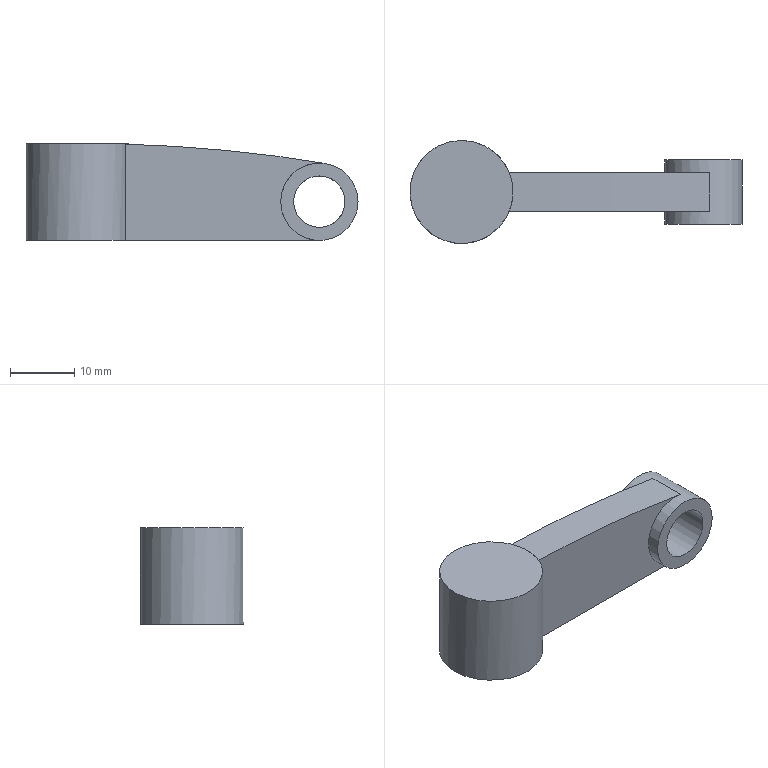Component | NX | CONNECTING_ROD_1 | 1 solid | 12 faces | box 51.54 x 16 x 15 mm | volume 4830 mm3 | plane 7 | cylinder 5 | commonest cylinder face diameters 16 x1 447 x1 12 x1 10 x1 8 x1
STEP:
#1=CARTESIAN_POINT('',(0.,0.,0.));
#2=DIRECTION('',(0.,0.,1.));
#3=DIRECTION('',(1.,0.,0.));
#4=AXIS2_PLACEMENT_3D('',#1,#2,#3);
#5=CARTESIAN_POINT('',(-285.764,8.,132.303));
#6=VERTEX_POINT('',#5);
#7=CARTESIAN_POINT('',(-285.764,0.,132.303));
#8=DIRECTION('',(0.,0.,-1.));
#9=DIRECTION('',(0.,1.,0.));
#10=AXIS2_PLACEMENT_3D('',#7,#8,#9);
#11=CIRCLE('',#10,8.);
#12=CARTESIAN_POINT('',(-285.764,0.,117.303));
#13=DIRECTION('',(0.,0.,1.));
#14=DIRECTION('',(0.,1.,0.));
#15=AXIS2_PLACEMENT_3D('',#12,#13,#14);
#16=CYLINDRICAL_SURFACE('',#15,8.);
#17=CARTESIAN_POINT('',(6.283,15.));
#18=DIRECTION('',(-1.,0.));
#19=VECTOR('',#18,1.);
#20=LINE('',#17,#19);
#21=(GEOMETRIC_REPRESENTATION_CONTEXT(2)PARAMETRIC_REPRESENTATION_CONTEXT()REPRESENTATION_CONTEXT('',''));
#22=DEFINITIONAL_REPRESENTATION('',(#20),#21);
#23=PCURVE('',#16,#22);
#24=CARTESIAN_POINT('',(-285.764,0.,132.303));
#25=DIRECTION('',(0.,0.,1.));
#26=DIRECTION('',(0.,1.,0.));
#27=AXIS2_PLACEMENT_3D('',#24,#25,#26);
#28=PLANE('',#27);
#29=CARTESIAN_POINT('',(8.,0.));
#30=CARTESIAN_POINT('',(8.,-13.856));
#31=CARTESIAN_POINT('',(-4.,-6.928));
#32=CARTESIAN_POINT('',(-16.,-0.));
#33=CARTESIAN_POINT('',(-4.,6.928));
#34=CARTESIAN_POINT('',(8.,13.856));
#35=CARTESIAN_POINT('',(8.,0.));
#36=(BOUNDED_CURVE()B_SPLINE_CURVE(2,(#29,#30,#31,#32,#33,#34,#35),.UNSPECIFIED.,.T.,.F.)B_SPLINE_CURVE_WITH_KNOTS((1,2,2,2,2,1),(-2.094,0.,2.094,4.189,6.283,8.378),.UNSPECIFIED.)CURVE()GEOMETRIC_REPRESENTATION_ITEM()RATIONAL_B_SPLINE_CURVE((1.,0.5,1.,0.5,1.,0.5,1.))REPRESENTATION_ITEM(''));
#37=(GEOMETRIC_REPRESENTATION_CONTEXT(2)PARAMETRIC_REPRESENTATION_CONTEXT()REPRESENTATION_CONTEXT('',''));
#38=DEFINITIONAL_REPRESENTATION('',(#36),#37);
#39=PCURVE('',#28,#38);
#40=SURFACE_CURVE('',#11,(#23,#39),.PCURVE_S1.);
#41=EDGE_CURVE('',#6,#6,#40,.T.);
#42=ORIENTED_EDGE('',*,*,#41,.T.);
#43=CARTESIAN_POINT('',(-285.764,8.,117.303));
#44=VERTEX_POINT('',#43);
#45=CARTESIAN_POINT('',(-285.764,8.,117.303));
#46=CARTESIAN_POINT('',(-285.764,8.,132.303));
#47=B_SPLINE_CURVE_WITH_KNOTS('',1,(#45,#46),.UNSPECIFIED.,.F.,.F.,(2,2),(0.,15.),.PIECEWISE_BEZIER_KNOTS.);
#48=CARTESIAN_POINT('',(0.,0.));
#49=DIRECTION('',(0.,1.));
#50=VECTOR('',#49,1.);
#51=LINE('',#48,#50);
#52=(GEOMETRIC_REPRESENTATION_CONTEXT(2)PARAMETRIC_REPRESENTATION_CONTEXT()REPRESENTATION_CONTEXT('',''));
#53=DEFINITIONAL_REPRESENTATION('',(#51),#52);
#54=PCURVE('',#16,#53);
#55=CARTESIAN_POINT('',(6.283,0.));
#56=DIRECTION('',(0.,1.));
#57=VECTOR('',#56,1.);
#58=LINE('',#55,#57);
#59=(GEOMETRIC_REPRESENTATION_CONTEXT(2)PARAMETRIC_REPRESENTATION_CONTEXT()REPRESENTATION_CONTEXT('',''));
#60=DEFINITIONAL_REPRESENTATION('',(#58),#59);
#61=PCURVE('',#16,#60);
#62=SEAM_CURVE('',#47,(#54,#61),.PCURVE_S1.);
#63=EDGE_CURVE('',#44,#6,#62,.T.);
#64=ORIENTED_EDGE('',*,*,#63,.F.);
#65=CARTESIAN_POINT('',(-278.348,-3.,117.303));
#66=VERTEX_POINT('',#65);
#67=CARTESIAN_POINT('',(-285.764,0.,117.303));
#68=DIRECTION('',(0.,0.,1.));
#69=DIRECTION('',(0.,1.,0.));
#70=AXIS2_PLACEMENT_3D('',#67,#68,#69);
#71=CIRCLE('',#70,8.);
#72=CARTESIAN_POINT('',(-0.,0.));
#73=DIRECTION('',(1.,0.));
#74=VECTOR('',#73,1.);
#75=LINE('',#72,#74);
#76=(GEOMETRIC_REPRESENTATION_CONTEXT(2)PARAMETRIC_REPRESENTATION_CONTEXT()REPRESENTATION_CONTEXT('',''));
#77=DEFINITIONAL_REPRESENTATION('',(#75),#76);
#78=PCURVE('',#16,#77);
#79=CARTESIAN_POINT('',(-285.764,0.,117.303));
#80=DIRECTION('',(0.,0.,-1.));
#81=DIRECTION('',(0.,-1.,0.));
#82=AXIS2_PLACEMENT_3D('',#79,#80,#81);
#83=PLANE('',#82);
#84=CARTESIAN_POINT('',(-8.,0.));
#85=CARTESIAN_POINT('',(-8.,13.856));
#86=CARTESIAN_POINT('',(4.,6.928));
#87=CARTESIAN_POINT('',(16.,0.));
#88=CARTESIAN_POINT('',(4.,-6.928));
#89=CARTESIAN_POINT('',(-8.,-13.856));
#90=CARTESIAN_POINT('',(-8.,0.));
#91=(BOUNDED_CURVE()B_SPLINE_CURVE(2,(#84,#85,#86,#87,#88,#89,#90),.UNSPECIFIED.,.T.,.F.)B_SPLINE_CURVE_WITH_KNOTS((1,2,2,2,2,1),(-2.094,0.,2.094,4.189,6.283,8.378),.UNSPECIFIED.)CURVE()GEOMETRIC_REPRESENTATION_ITEM()RATIONAL_B_SPLINE_CURVE((1.,0.5,1.,0.5,1.,0.5,1.))REPRESENTATION_ITEM(''));
#92=(GEOMETRIC_REPRESENTATION_CONTEXT(2)PARAMETRIC_REPRESENTATION_CONTEXT()REPRESENTATION_CONTEXT('',''));
#93=DEFINITIONAL_REPRESENTATION('',(#91),#92);
#94=PCURVE('',#83,#93);
#95=SURFACE_CURVE('',#71,(#78,#94),.PCURVE_S1.);
#96=EDGE_CURVE('',#44,#66,#95,.T.);
#97=ORIENTED_EDGE('',*,*,#96,.T.);
#98=CARTESIAN_POINT('',(-278.348,-3.,132.226));
#99=VERTEX_POINT('',#98);
#100=CARTESIAN_POINT('',(-278.348,-3.,117.303));
#101=DIRECTION('',(0.,0.,-1.));
#102=VECTOR('',#101,1.);
#103=LINE('',#100,#102);
#104=CARTESIAN_POINT('',(4.328,0.));
#105=DIRECTION('',(0.,-1.));
#106=VECTOR('',#105,1.);
#107=LINE('',#104,#106);
#108=(GEOMETRIC_REPRESENTATION_CONTEXT(2)PARAMETRIC_REPRESENTATION_CONTEXT()REPRESENTATION_CONTEXT('',''));
#109=DEFINITIONAL_REPRESENTATION('',(#107),#108);
#110=PCURVE('',#16,#109);
#111=CARTESIAN_POINT('',(-248.225,-3.,123.303));
#112=DIRECTION('',(0.,-1.,0.));
#113=DIRECTION('',(0.,0.,1.));
#114=AXIS2_PLACEMENT_3D('',#111,#112,#113);
#115=PLANE('',#114);
#116=CARTESIAN_POINT('',(-6.,30.123));
#117=DIRECTION('',(-1.,0.));
#118=VECTOR('',#117,1.);
#119=LINE('',#116,#118);
#120=(GEOMETRIC_REPRESENTATION_CONTEXT(2)PARAMETRIC_REPRESENTATION_CONTEXT()REPRESENTATION_CONTEXT('',''));
#121=DEFINITIONAL_REPRESENTATION('',(#119),#120);
#122=PCURVE('',#115,#121);
#123=SURFACE_CURVE('',#103,(#110,#122),.PCURVE_S1.);
#124=EDGE_CURVE('',#99,#66,#123,.T.);
#125=ORIENTED_EDGE('',*,*,#124,.F.);
#126=CARTESIAN_POINT('',(-278.348,3.,132.226));
#127=VERTEX_POINT('',#126);
#128=CARTESIAN_POINT('',(-278.348,-3.,132.226));
#129=CARTESIAN_POINT('',(-277.573,-1.083,132.205));
#130=CARTESIAN_POINT('',(-277.573,1.083,132.205));
#131=CARTESIAN_POINT('',(-278.348,3.,132.226));
#132=B_SPLINE_CURVE_WITH_KNOTS('',3,(#128,#129,#130,#131),.UNSPECIFIED.,.F.,.F.,(4,4),(0.,1.),.PIECEWISE_BEZIER_KNOTS.);
#133=CARTESIAN_POINT('',(4.328,14.923));
#134=CARTESIAN_POINT('',(5.097,14.923));
#135=B_SPLINE_CURVE_WITH_KNOTS('',1,(#133,#134),.UNSPECIFIED.,.F.,.F.,(2,2),(0.,1.),.PIECEWISE_BEZIER_KNOTS.);
#136=(GEOMETRIC_REPRESENTATION_CONTEXT(2)PARAMETRIC_REPRESENTATION_CONTEXT()REPRESENTATION_CONTEXT('',''));
#137=DEFINITIONAL_REPRESENTATION('',(#135),#136);
#138=PCURVE('',#16,#137);
#139=CARTESIAN_POINT('',(-284.225,3.,-91.197));
#140=DIRECTION('',(0.,-1.,0.));
#141=DIRECTION('',(0.,0.,1.));
#142=AXIS2_PLACEMENT_3D('',#139,#140,#141);
#143=CYLINDRICAL_SURFACE('',#142,223.5);
#144=CARTESIAN_POINT('',(6.257,6.));
#145=CARTESIAN_POINT('',(6.257,5.913));
#146=CARTESIAN_POINT('',(6.256,5.738));
#147=CARTESIAN_POINT('',(6.256,5.472));
#148=CARTESIAN_POINT('',(6.256,5.204));
#149=CARTESIAN_POINT('',(6.255,4.933));
#150=CARTESIAN_POINT('',(6.255,4.661));
#151=CARTESIAN_POINT('',(6.255,4.386));
#152=CARTESIAN_POINT('',(6.255,4.111));
#153=CARTESIAN_POINT('',(6.254,3.834));
#154=CARTESIAN_POINT('',(6.254,3.557));
#155=CARTESIAN_POINT('',(6.254,3.278));
#156=CARTESIAN_POINT('',(6.254,3.));
#157=CARTESIAN_POINT('',(6.254,2.722));
#158=CARTESIAN_POINT('',(6.254,2.443));
#159=CARTESIAN_POINT('',(6.254,2.166));
#160=CARTESIAN_POINT('',(6.255,1.889));
#161=CARTESIAN_POINT('',(6.255,1.614));
#162=CARTESIAN_POINT('',(6.255,1.339));
#163=CARTESIAN_POINT('',(6.255,1.067));
#164=CARTESIAN_POINT('',(6.256,0.7964));
#165=CARTESIAN_POINT('',(6.256,0.5281));
#166=CARTESIAN_POINT('',(6.256,0.2624));
#167=CARTESIAN_POINT('',(6.257,0.08712));
#168=CARTESIAN_POINT('',(6.257,0.));
#169=B_SPLINE_CURVE_WITH_KNOTS('',3,(#144,#145,#146,#147,#148,#149,#150,#151,#152,#153,#154,#155,#156,#157,#158,#159,#160,#161,#162,#163,#164,#165,#166,#167,#168),.UNSPECIFIED.,.F.,.F.,(4,1,1,1,1,1,1,1,1,1,1,1,1,1,1,1,1,1,1,1,1,1,4),(0.,0.04545,0.09091,0.1364,0.1818,0.2273,0.2727,0.3182,0.3636,0.4091,0.4545,0.5,0.5455,0.5909,0.6364,0.6818,0.7273,0.7727,0.8182,0.8636,0.9091,0.9545,1.),.QUASI_UNIFORM_KNOTS.);
#170=(GEOMETRIC_REPRESENTATION_CONTEXT(2)PARAMETRIC_REPRESENTATION_CONTEXT()REPRESENTATION_CONTEXT('',''));
#171=DEFINITIONAL_REPRESENTATION('',(#169),#170);
#172=PCURVE('',#143,#171);
#173=SURFACE_CURVE('',#132,(#138,#172),.PCURVE_S1.);
#174=EDGE_CURVE('',#99,#127,#173,.T.);
#175=ORIENTED_EDGE('',*,*,#174,.T.);
#176=CARTESIAN_POINT('',(-278.348,3.,117.303));
#177=VERTEX_POINT('',#176);
#178=CARTESIAN_POINT('',(-278.348,3.,117.303));
#179=DIRECTION('',(0.,0.,-1.));
#180=VECTOR('',#179,1.);
#181=LINE('',#178,#180);
#182=CARTESIAN_POINT('',(5.097,0.));
#183=DIRECTION('',(0.,-1.));
#184=VECTOR('',#183,1.);
#185=LINE('',#182,#184);
#186=(GEOMETRIC_REPRESENTATION_CONTEXT(2)PARAMETRIC_REPRESENTATION_CONTEXT()REPRESENTATION_CONTEXT('',''));
#187=DEFINITIONAL_REPRESENTATION('',(#185),#186);
#188=PCURVE('',#16,#187);
#189=CARTESIAN_POINT('',(-248.225,3.,123.303));
#190=DIRECTION('',(0.,-1.,0.));
#191=DIRECTION('',(0.,0.,1.));
#192=AXIS2_PLACEMENT_3D('',#189,#190,#191);
#193=PLANE('',#192);
#194=CARTESIAN_POINT('',(-6.,30.123));
#195=DIRECTION('',(-1.,0.));
#196=VECTOR('',#195,1.);
#197=LINE('',#194,#196);
#198=(GEOMETRIC_REPRESENTATION_CONTEXT(2)PARAMETRIC_REPRESENTATION_CONTEXT()REPRESENTATION_CONTEXT('',''));
#199=DEFINITIONAL_REPRESENTATION('',(#197),#198);
#200=PCURVE('',#193,#199);
#201=SURFACE_CURVE('',#181,(#188,#200),.PCURVE_S1.);
#202=EDGE_CURVE('',#127,#177,#201,.T.);
#203=ORIENTED_EDGE('',*,*,#202,.T.);
#204=CARTESIAN_POINT('',(-285.764,0.,117.303));
#205=DIRECTION('',(0.,0.,1.));
#206=DIRECTION('',(0.,1.,0.));
#207=AXIS2_PLACEMENT_3D('',#204,#205,#206);
#208=CIRCLE('',#207,8.);
#209=CARTESIAN_POINT('',(-0.,0.));
#210=DIRECTION('',(1.,0.));
#211=VECTOR('',#210,1.);
#212=LINE('',#209,#211);
#213=(GEOMETRIC_REPRESENTATION_CONTEXT(2)PARAMETRIC_REPRESENTATION_CONTEXT()REPRESENTATION_CONTEXT('',''));
#214=DEFINITIONAL_REPRESENTATION('',(#212),#213);
#215=PCURVE('',#16,#214);
#216=CARTESIAN_POINT('',(-8.,0.));
#217=CARTESIAN_POINT('',(-8.,13.856));
#218=CARTESIAN_POINT('',(4.,6.928));
#219=CARTESIAN_POINT('',(16.,0.));
#220=CARTESIAN_POINT('',(4.,-6.928));
#221=CARTESIAN_POINT('',(-8.,-13.856));
#222=CARTESIAN_POINT('',(-8.,0.));
#223=(BOUNDED_CURVE()B_SPLINE_CURVE(2,(#216,#217,#218,#219,#220,#221,#222),.UNSPECIFIED.,.T.,.F.)B_SPLINE_CURVE_WITH_KNOTS((1,2,2,2,2,1),(-2.094,0.,2.094,4.189,6.283,8.378),.UNSPECIFIED.)CURVE()GEOMETRIC_REPRESENTATION_ITEM()RATIONAL_B_SPLINE_CURVE((1.,0.5,1.,0.5,1.,0.5,1.))REPRESENTATION_ITEM(''));
#224=(GEOMETRIC_REPRESENTATION_CONTEXT(2)PARAMETRIC_REPRESENTATION_CONTEXT()REPRESENTATION_CONTEXT('',''));
#225=DEFINITIONAL_REPRESENTATION('',(#223),#224);
#226=PCURVE('',#83,#225);
#227=SURFACE_CURVE('',#208,(#215,#226),.PCURVE_S1.);
#228=EDGE_CURVE('',#177,#44,#227,.T.);
#229=ORIENTED_EDGE('',*,*,#228,.T.);
#230=ORIENTED_EDGE('',*,*,#63,.T.);
#231=EDGE_LOOP('',(#42,#64,#97,#125,#175,#203,#229,#230));
#232=FACE_BOUND('',#231,.T.);
#233=ADVANCED_FACE('',(#232),#16,.T.);
#234=ORIENTED_EDGE('',*,*,#41,.F.);
#235=EDGE_LOOP('',(#234));
#236=FACE_BOUND('',#235,.T.);
#237=ADVANCED_FACE('',(#236),#28,.T.);
#238=CARTESIAN_POINT('',(-290.764,0.,117.303));
#239=VERTEX_POINT('',#238);
#240=CARTESIAN_POINT('',(-285.764,0.,117.303));
#241=DIRECTION('',(0.,0.,-1.));
#242=DIRECTION('',(-1.,-0.,0.));
#243=AXIS2_PLACEMENT_3D('',#240,#241,#242);
#244=CIRCLE('',#243,5.);
#245=CARTESIAN_POINT('',(0.,0.));
#246=DIRECTION('',(0.,1.));
#247=AXIS2_PLACEMENT_2D('',#245,#246);
#248=CIRCLE('',#247,5.);
#249=(GEOMETRIC_REPRESENTATION_CONTEXT(2)PARAMETRIC_REPRESENTATION_CONTEXT()REPRESENTATION_CONTEXT('',''));
#250=DEFINITIONAL_REPRESENTATION('',(#248),#249);
#251=PCURVE('',#83,#250);
#252=CARTESIAN_POINT('',(-285.764,0.,129.303));
#253=DIRECTION('',(0.,0.,-1.));
#254=DIRECTION('',(0.,-1.,0.));
#255=AXIS2_PLACEMENT_3D('',#252,#253,#254);
#256=CYLINDRICAL_SURFACE('',#255,5.);
#257=CARTESIAN_POINT('',(1.571,12.));
#258=DIRECTION('',(1.,0.));
#259=VECTOR('',#258,1.);
#260=LINE('',#257,#259);
#261=(GEOMETRIC_REPRESENTATION_CONTEXT(2)PARAMETRIC_REPRESENTATION_CONTEXT()REPRESENTATION_CONTEXT('',''));
#262=DEFINITIONAL_REPRESENTATION('',(#260),#261);
#263=PCURVE('',#256,#262);
#264=SURFACE_CURVE('',#244,(#251,#263),.PCURVE_S1.);
#265=EDGE_CURVE('',#239,#239,#264,.T.);
#266=ORIENTED_EDGE('',*,*,#265,.F.);
#267=EDGE_LOOP('',(#266));
#268=FACE_BOUND('',#267,.T.);
#269=ORIENTED_EDGE('',*,*,#228,.F.);
#270=CARTESIAN_POINT('',(-248.225,3.,117.303));
#271=VERTEX_POINT('',#270);
#272=CARTESIAN_POINT('',(-248.225,3.,117.303));
#273=DIRECTION('',(-1.,0.,0.));
#274=VECTOR('',#273,1.);
#275=LINE('',#272,#274);
#276=CARTESIAN_POINT('',(-3.,-37.539));
#277=DIRECTION('',(0.,1.));
#278=VECTOR('',#277,1.);
#279=LINE('',#276,#278);
#280=(GEOMETRIC_REPRESENTATION_CONTEXT(2)PARAMETRIC_REPRESENTATION_CONTEXT()REPRESENTATION_CONTEXT('',''));
#281=DEFINITIONAL_REPRESENTATION('',(#279),#280);
#282=PCURVE('',#83,#281);
#283=CARTESIAN_POINT('',(-6.,0.));
#284=DIRECTION('',(0.,1.));
#285=VECTOR('',#284,1.);
#286=LINE('',#283,#285);
#287=(GEOMETRIC_REPRESENTATION_CONTEXT(2)PARAMETRIC_REPRESENTATION_CONTEXT()REPRESENTATION_CONTEXT('',''));
#288=DEFINITIONAL_REPRESENTATION('',(#286),#287);
#289=PCURVE('',#193,#288);
#290=SURFACE_CURVE('',#275,(#282,#289),.PCURVE_S1.);
#291=EDGE_CURVE('',#271,#177,#290,.T.);
#292=ORIENTED_EDGE('',*,*,#291,.F.);
#293=CARTESIAN_POINT('',(-248.225,-3.,117.303));
#294=VERTEX_POINT('',#293);
#295=CARTESIAN_POINT('',(-248.225,3.,117.303));
#296=DIRECTION('',(0.,-1.,0.));
#297=VECTOR('',#296,1.);
#298=LINE('',#295,#297);
#299=CARTESIAN_POINT('',(-3.,-37.539));
#300=DIRECTION('',(1.,0.));
#301=VECTOR('',#300,1.);
#302=LINE('',#299,#301);
#303=(GEOMETRIC_REPRESENTATION_CONTEXT(2)PARAMETRIC_REPRESENTATION_CONTEXT()REPRESENTATION_CONTEXT('',''));
#304=DEFINITIONAL_REPRESENTATION('',(#302),#303);
#305=PCURVE('',#83,#304);
#306=CARTESIAN_POINT('',(-248.225,5.,123.303));
#307=DIRECTION('',(0.,-1.,0.));
#308=DIRECTION('',(0.,0.,1.));
#309=AXIS2_PLACEMENT_3D('',#306,#307,#308);
#310=CYLINDRICAL_SURFACE('',#309,6.);
#311=CARTESIAN_POINT('',(3.142,2.));
#312=DIRECTION('',(0.,1.));
#313=VECTOR('',#312,1.);
#314=LINE('',#311,#313);
#315=(GEOMETRIC_REPRESENTATION_CONTEXT(2)PARAMETRIC_REPRESENTATION_CONTEXT()REPRESENTATION_CONTEXT('',''));
#316=DEFINITIONAL_REPRESENTATION('',(#314),#315);
#317=PCURVE('',#310,#316);
#318=SURFACE_CURVE('',#298,(#305,#317),.PCURVE_S1.);
#319=EDGE_CURVE('',#271,#294,#318,.T.);
#320=ORIENTED_EDGE('',*,*,#319,.T.);
#321=CARTESIAN_POINT('',(-248.225,-3.,117.303));
#322=DIRECTION('',(-1.,0.,0.));
#323=VECTOR('',#322,1.);
#324=LINE('',#321,#323);
#325=CARTESIAN_POINT('',(3.,-37.539));
#326=DIRECTION('',(0.,1.));
#327=VECTOR('',#326,1.);
#328=LINE('',#325,#327);
#329=(GEOMETRIC_REPRESENTATION_CONTEXT(2)PARAMETRIC_REPRESENTATION_CONTEXT()REPRESENTATION_CONTEXT('',''));
#330=DEFINITIONAL_REPRESENTATION('',(#328),#329);
#331=PCURVE('',#83,#330);
#332=CARTESIAN_POINT('',(-6.,0.));
#333=DIRECTION('',(0.,1.));
#334=VECTOR('',#333,1.);
#335=LINE('',#332,#334);
#336=(GEOMETRIC_REPRESENTATION_CONTEXT(2)PARAMETRIC_REPRESENTATION_CONTEXT()REPRESENTATION_CONTEXT('',''));
#337=DEFINITIONAL_REPRESENTATION('',(#335),#336);
#338=PCURVE('',#115,#337);
#339=SURFACE_CURVE('',#324,(#331,#338),.PCURVE_S1.);
#340=EDGE_CURVE('',#294,#66,#339,.T.);
#341=ORIENTED_EDGE('',*,*,#340,.T.);
#342=ORIENTED_EDGE('',*,*,#96,.F.);
#343=EDGE_LOOP('',(#269,#292,#320,#341,#342));
#344=FACE_BOUND('',#343,.T.);
#345=ADVANCED_FACE('',(#268,#344),#83,.T.);
#346=ORIENTED_EDGE('',*,*,#174,.F.);
#347=CARTESIAN_POINT('',(-247.232,-3.,129.22));
#348=VERTEX_POINT('',#347);
#349=CARTESIAN_POINT('',(-284.225,-3.,-91.197));
#350=DIRECTION('',(0.,1.,0.));
#351=DIRECTION('',(-1.,0.,-0.));
#352=AXIS2_PLACEMENT_3D('',#349,#350,#351);
#353=CIRCLE('',#352,223.5);
#354=CARTESIAN_POINT('',(7.854,6.));
#355=DIRECTION('',(-1.,0.));
#356=VECTOR('',#355,1.);
#357=LINE('',#354,#356);
#358=(GEOMETRIC_REPRESENTATION_CONTEXT(2)PARAMETRIC_REPRESENTATION_CONTEXT()REPRESENTATION_CONTEXT('',''));
#359=DEFINITIONAL_REPRESENTATION('',(#357),#358);
#360=PCURVE('',#143,#359);
#361=CARTESIAN_POINT('',(-214.5,259.5));
#362=CARTESIAN_POINT('',(172.613,259.5));
#363=CARTESIAN_POINT('',(-20.943,-75.75));
#364=CARTESIAN_POINT('',(-214.5,-411.));
#365=CARTESIAN_POINT('',(-408.057,-75.75));
#366=CARTESIAN_POINT('',(-601.613,259.5));
#367=CARTESIAN_POINT('',(-214.5,259.5));
#368=(BOUNDED_CURVE()B_SPLINE_CURVE(2,(#361,#362,#363,#364,#365,#366,#367),.UNSPECIFIED.,.T.,.F.)B_SPLINE_CURVE_WITH_KNOTS((1,2,2,2,2,1),(-2.094,0.,2.094,4.189,6.283,8.378),.UNSPECIFIED.)CURVE()GEOMETRIC_REPRESENTATION_ITEM()RATIONAL_B_SPLINE_CURVE((1.,0.5,1.,0.5,1.,0.5,1.))REPRESENTATION_ITEM(''));
#369=(GEOMETRIC_REPRESENTATION_CONTEXT(2)PARAMETRIC_REPRESENTATION_CONTEXT()REPRESENTATION_CONTEXT('',''));
#370=DEFINITIONAL_REPRESENTATION('',(#368),#369);
#371=PCURVE('',#115,#370);
#372=SURFACE_CURVE('',#353,(#360,#371),.PCURVE_S1.);
#373=EDGE_CURVE('',#99,#348,#372,.T.);
#374=ORIENTED_EDGE('',*,*,#373,.T.);
#375=CARTESIAN_POINT('',(-247.232,3.,129.22));
#376=VERTEX_POINT('',#375);
#377=CARTESIAN_POINT('',(-247.232,3.,129.22));
#378=DIRECTION('',(0.,-1.,0.));
#379=VECTOR('',#378,1.);
#380=LINE('',#377,#379);
#381=CARTESIAN_POINT('',(6.117,0.));
#382=DIRECTION('',(0.,1.));
#383=VECTOR('',#382,1.);
#384=LINE('',#381,#383);
#385=(GEOMETRIC_REPRESENTATION_CONTEXT(2)PARAMETRIC_REPRESENTATION_CONTEXT()REPRESENTATION_CONTEXT('',''));
#386=DEFINITIONAL_REPRESENTATION('',(#384),#385);
#387=PCURVE('',#143,#386);
#388=CARTESIAN_POINT('',(6.117,2.));
#389=DIRECTION('',(0.,1.));
#390=VECTOR('',#389,1.);
#391=LINE('',#388,#390);
#392=(GEOMETRIC_REPRESENTATION_CONTEXT(2)PARAMETRIC_REPRESENTATION_CONTEXT()REPRESENTATION_CONTEXT('',''));
#393=DEFINITIONAL_REPRESENTATION('',(#391),#392);
#394=PCURVE('',#310,#393);
#395=SURFACE_CURVE('',#380,(#387,#394),.PCURVE_S1.);
#396=EDGE_CURVE('',#376,#348,#395,.T.);
#397=ORIENTED_EDGE('',*,*,#396,.F.);
#398=CARTESIAN_POINT('',(-284.225,3.,-91.197));
#399=DIRECTION('',(0.,1.,0.));
#400=DIRECTION('',(-1.,0.,-0.));
#401=AXIS2_PLACEMENT_3D('',#398,#399,#400);
#402=CIRCLE('',#401,223.5);
#403=CARTESIAN_POINT('',(7.854,0.));
#404=DIRECTION('',(-1.,0.));
#405=VECTOR('',#404,1.);
#406=LINE('',#403,#405);
#407=(GEOMETRIC_REPRESENTATION_CONTEXT(2)PARAMETRIC_REPRESENTATION_CONTEXT()REPRESENTATION_CONTEXT('',''));
#408=DEFINITIONAL_REPRESENTATION('',(#406),#407);
#409=PCURVE('',#143,#408);
#410=CARTESIAN_POINT('',(-214.5,259.5));
#411=CARTESIAN_POINT('',(172.613,259.5));
#412=CARTESIAN_POINT('',(-20.943,-75.75));
#413=CARTESIAN_POINT('',(-214.5,-411.));
#414=CARTESIAN_POINT('',(-408.057,-75.75));
#415=CARTESIAN_POINT('',(-601.613,259.5));
#416=CARTESIAN_POINT('',(-214.5,259.5));
#417=(BOUNDED_CURVE()B_SPLINE_CURVE(2,(#410,#411,#412,#413,#414,#415,#416),.UNSPECIFIED.,.T.,.F.)B_SPLINE_CURVE_WITH_KNOTS((1,2,2,2,2,1),(-2.094,0.,2.094,4.189,6.283,8.378),.UNSPECIFIED.)CURVE()GEOMETRIC_REPRESENTATION_ITEM()RATIONAL_B_SPLINE_CURVE((1.,0.5,1.,0.5,1.,0.5,1.))REPRESENTATION_ITEM(''));
#418=(GEOMETRIC_REPRESENTATION_CONTEXT(2)PARAMETRIC_REPRESENTATION_CONTEXT()REPRESENTATION_CONTEXT('',''));
#419=DEFINITIONAL_REPRESENTATION('',(#417),#418);
#420=PCURVE('',#193,#419);
#421=SURFACE_CURVE('',#402,(#409,#420),.PCURVE_S1.);
#422=EDGE_CURVE('',#127,#376,#421,.T.);
#423=ORIENTED_EDGE('',*,*,#422,.F.);
#424=EDGE_LOOP('',(#346,#374,#397,#423));
#425=FACE_BOUND('',#424,.T.);
#426=ADVANCED_FACE('',(#425),#143,.T.);
#427=ORIENTED_EDGE('',*,*,#202,.F.);
#428=ORIENTED_EDGE('',*,*,#422,.T.);
#429=CARTESIAN_POINT('',(-254.225,3.,123.303));
#430=VERTEX_POINT('',#429);
#431=CARTESIAN_POINT('',(-248.225,3.,123.303));
#432=DIRECTION('',(0.,-1.,0.));
#433=DIRECTION('',(-1.,0.,0.));
#434=AXIS2_PLACEMENT_3D('',#431,#432,#433);
#435=CIRCLE('',#434,6.);
#436=CARTESIAN_POINT('',(0.,0.));
#437=DIRECTION('',(0.,1.));
#438=AXIS2_PLACEMENT_2D('',#436,#437);
#439=CIRCLE('',#438,6.);
#440=(GEOMETRIC_REPRESENTATION_CONTEXT(2)PARAMETRIC_REPRESENTATION_CONTEXT()REPRESENTATION_CONTEXT('',''));
#441=DEFINITIONAL_REPRESENTATION('',(#439),#440);
#442=PCURVE('',#193,#441);
#443=CARTESIAN_POINT('',(1.571,2.));
#444=DIRECTION('',(1.,0.));
#445=VECTOR('',#444,1.);
#446=LINE('',#443,#445);
#447=(GEOMETRIC_REPRESENTATION_CONTEXT(2)PARAMETRIC_REPRESENTATION_CONTEXT()REPRESENTATION_CONTEXT('',''));
#448=DEFINITIONAL_REPRESENTATION('',(#446),#447);
#449=PCURVE('',#310,#448);
#450=SURFACE_CURVE('',#435,(#442,#449),.PCURVE_S1.);
#451=EDGE_CURVE('',#376,#430,#450,.T.);
#452=ORIENTED_EDGE('',*,*,#451,.T.);
#453=CARTESIAN_POINT('',(-248.225,3.,123.303));
#454=DIRECTION('',(0.,-1.,0.));
#455=DIRECTION('',(-1.,0.,0.));
#456=AXIS2_PLACEMENT_3D('',#453,#454,#455);
#457=CIRCLE('',#456,6.);
#458=CARTESIAN_POINT('',(0.,0.));
#459=DIRECTION('',(0.,1.));
#460=AXIS2_PLACEMENT_2D('',#458,#459);
#461=CIRCLE('',#460,6.);
#462=(GEOMETRIC_REPRESENTATION_CONTEXT(2)PARAMETRIC_REPRESENTATION_CONTEXT()REPRESENTATION_CONTEXT('',''));
#463=DEFINITIONAL_REPRESENTATION('',(#461),#462);
#464=PCURVE('',#193,#463);
#465=CARTESIAN_POINT('',(-4.712,2.));
#466=DIRECTION('',(1.,0.));
#467=VECTOR('',#466,1.);
#468=LINE('',#465,#467);
#469=(GEOMETRIC_REPRESENTATION_CONTEXT(2)PARAMETRIC_REPRESENTATION_CONTEXT()REPRESENTATION_CONTEXT('',''));
#470=DEFINITIONAL_REPRESENTATION('',(#468),#469);
#471=PCURVE('',#310,#470);
#472=SURFACE_CURVE('',#457,(#464,#471),.PCURVE_S1.);
#473=EDGE_CURVE('',#430,#271,#472,.T.);
#474=ORIENTED_EDGE('',*,*,#473,.T.);
#475=ORIENTED_EDGE('',*,*,#291,.T.);
#476=EDGE_LOOP('',(#427,#428,#452,#474,#475));
#477=FACE_BOUND('',#476,.T.);
#478=ADVANCED_FACE('',(#477),#193,.F.);
#479=ORIENTED_EDGE('',*,*,#373,.F.);
#480=ORIENTED_EDGE('',*,*,#124,.T.);
#481=ORIENTED_EDGE('',*,*,#340,.F.);
#482=CARTESIAN_POINT('',(-254.225,-3.,123.303));
#483=VERTEX_POINT('',#482);
#484=CARTESIAN_POINT('',(-248.225,-3.,123.303));
#485=DIRECTION('',(0.,-1.,0.));
#486=DIRECTION('',(-1.,0.,0.));
#487=AXIS2_PLACEMENT_3D('',#484,#485,#486);
#488=CIRCLE('',#487,6.);
#489=CARTESIAN_POINT('',(0.,0.));
#490=DIRECTION('',(0.,1.));
#491=AXIS2_PLACEMENT_2D('',#489,#490);
#492=CIRCLE('',#491,6.);
#493=(GEOMETRIC_REPRESENTATION_CONTEXT(2)PARAMETRIC_REPRESENTATION_CONTEXT()REPRESENTATION_CONTEXT('',''));
#494=DEFINITIONAL_REPRESENTATION('',(#492),#493);
#495=PCURVE('',#115,#494);
#496=CARTESIAN_POINT('',(-4.712,8.));
#497=DIRECTION('',(1.,0.));
#498=VECTOR('',#497,1.);
#499=LINE('',#496,#498);
#500=(GEOMETRIC_REPRESENTATION_CONTEXT(2)PARAMETRIC_REPRESENTATION_CONTEXT()REPRESENTATION_CONTEXT('',''));
#501=DEFINITIONAL_REPRESENTATION('',(#499),#500);
#502=PCURVE('',#310,#501);
#503=SURFACE_CURVE('',#488,(#495,#502),.PCURVE_S1.);
#504=EDGE_CURVE('',#483,#294,#503,.T.);
#505=ORIENTED_EDGE('',*,*,#504,.F.);
#506=CARTESIAN_POINT('',(-248.225,-3.,123.303));
#507=DIRECTION('',(0.,-1.,0.));
#508=DIRECTION('',(-1.,0.,0.));
#509=AXIS2_PLACEMENT_3D('',#506,#507,#508);
#510=CIRCLE('',#509,6.);
#511=CARTESIAN_POINT('',(0.,0.));
#512=DIRECTION('',(0.,1.));
#513=AXIS2_PLACEMENT_2D('',#511,#512);
#514=CIRCLE('',#513,6.);
#515=(GEOMETRIC_REPRESENTATION_CONTEXT(2)PARAMETRIC_REPRESENTATION_CONTEXT()REPRESENTATION_CONTEXT('',''));
#516=DEFINITIONAL_REPRESENTATION('',(#514),#515);
#517=PCURVE('',#115,#516);
#518=CARTESIAN_POINT('',(1.571,8.));
#519=DIRECTION('',(1.,0.));
#520=VECTOR('',#519,1.);
#521=LINE('',#518,#520);
#522=(GEOMETRIC_REPRESENTATION_CONTEXT(2)PARAMETRIC_REPRESENTATION_CONTEXT()REPRESENTATION_CONTEXT('',''));
#523=DEFINITIONAL_REPRESENTATION('',(#521),#522);
#524=PCURVE('',#310,#523);
#525=SURFACE_CURVE('',#510,(#517,#524),.PCURVE_S1.);
#526=EDGE_CURVE('',#348,#483,#525,.T.);
#527=ORIENTED_EDGE('',*,*,#526,.F.);
#528=EDGE_LOOP('',(#479,#480,#481,#505,#527));
#529=FACE_BOUND('',#528,.T.);
#530=ADVANCED_FACE('',(#529),#115,.T.);
#531=ORIENTED_EDGE('',*,*,#319,.F.);
#532=ORIENTED_EDGE('',*,*,#473,.F.);
#533=CARTESIAN_POINT('',(-254.225,5.,123.303));
#534=VERTEX_POINT('',#533);
#535=CARTESIAN_POINT('',(-254.225,5.,123.303));
#536=CARTESIAN_POINT('',(-254.225,3.,123.303));
#537=B_SPLINE_CURVE_WITH_KNOTS('',1,(#535,#536),.UNSPECIFIED.,.F.,.F.,(2,2),(0.,2.),.PIECEWISE_BEZIER_KNOTS.);
#538=CARTESIAN_POINT('',(1.571,0.));
#539=DIRECTION('',(0.,1.));
#540=VECTOR('',#539,1.);
#541=LINE('',#538,#540);
#542=(GEOMETRIC_REPRESENTATION_CONTEXT(2)PARAMETRIC_REPRESENTATION_CONTEXT()REPRESENTATION_CONTEXT('',''));
#543=DEFINITIONAL_REPRESENTATION('',(#541),#542);
#544=PCURVE('',#310,#543);
#545=CARTESIAN_POINT('',(7.854,0.));
#546=DIRECTION('',(0.,1.));
#547=VECTOR('',#546,1.);
#548=LINE('',#545,#547);
#549=(GEOMETRIC_REPRESENTATION_CONTEXT(2)PARAMETRIC_REPRESENTATION_CONTEXT()REPRESENTATION_CONTEXT('',''));
#550=DEFINITIONAL_REPRESENTATION('',(#548),#549);
#551=PCURVE('',#310,#550);
#552=SEAM_CURVE('',#537,(#544,#551),.PCURVE_S1.);
#553=EDGE_CURVE('',#534,#430,#552,.T.);
#554=ORIENTED_EDGE('',*,*,#553,.F.);
#555=CARTESIAN_POINT('',(-248.225,5.,123.303));
#556=DIRECTION('',(0.,1.,0.));
#557=DIRECTION('',(-1.,0.,0.));
#558=AXIS2_PLACEMENT_3D('',#555,#556,#557);
#559=CIRCLE('',#558,6.);
#560=CARTESIAN_POINT('',(7.854,0.));
#561=DIRECTION('',(-1.,0.));
#562=VECTOR('',#561,1.);
#563=LINE('',#560,#562);
#564=(GEOMETRIC_REPRESENTATION_CONTEXT(2)PARAMETRIC_REPRESENTATION_CONTEXT()REPRESENTATION_CONTEXT('',''));
#565=DEFINITIONAL_REPRESENTATION('',(#563),#564);
#566=PCURVE('',#310,#565);
#567=CARTESIAN_POINT('',(-248.225,5.,123.303));
#568=DIRECTION('',(0.,1.,0.));
#569=DIRECTION('',(0.,0.,-1.));
#570=AXIS2_PLACEMENT_3D('',#567,#568,#569);
#571=PLANE('',#570);
#572=CARTESIAN_POINT('',(0.,0.));
#573=DIRECTION('',(0.,1.));
#574=AXIS2_PLACEMENT_2D('',#572,#573);
#575=CIRCLE('',#574,6.);
#576=(GEOMETRIC_REPRESENTATION_CONTEXT(2)PARAMETRIC_REPRESENTATION_CONTEXT()REPRESENTATION_CONTEXT('',''));
#577=DEFINITIONAL_REPRESENTATION('',(#575),#576);
#578=PCURVE('',#571,#577);
#579=SURFACE_CURVE('',#559,(#566,#578),.PCURVE_S1.);
#580=EDGE_CURVE('',#534,#534,#579,.T.);
#581=ORIENTED_EDGE('',*,*,#580,.F.);
#582=ORIENTED_EDGE('',*,*,#553,.T.);
#583=ORIENTED_EDGE('',*,*,#451,.F.);
#584=ORIENTED_EDGE('',*,*,#396,.T.);
#585=ORIENTED_EDGE('',*,*,#526,.T.);
#586=CARTESIAN_POINT('',(-254.225,-5.,123.303));
#587=VERTEX_POINT('',#586);
#588=CARTESIAN_POINT('',(-254.225,-3.,123.303));
#589=CARTESIAN_POINT('',(-254.225,-5.,123.303));
#590=B_SPLINE_CURVE_WITH_KNOTS('',1,(#588,#589),.UNSPECIFIED.,.F.,.F.,(2,2),(8.,10.),.PIECEWISE_BEZIER_KNOTS.);
#591=CARTESIAN_POINT('',(7.854,0.));
#592=DIRECTION('',(0.,1.));
#593=VECTOR('',#592,1.);
#594=LINE('',#591,#593);
#595=(GEOMETRIC_REPRESENTATION_CONTEXT(2)PARAMETRIC_REPRESENTATION_CONTEXT()REPRESENTATION_CONTEXT('',''));
#596=DEFINITIONAL_REPRESENTATION('',(#594),#595);
#597=PCURVE('',#310,#596);
#598=CARTESIAN_POINT('',(1.571,0.));
#599=DIRECTION('',(0.,1.));
#600=VECTOR('',#599,1.);
#601=LINE('',#598,#600);
#602=(GEOMETRIC_REPRESENTATION_CONTEXT(2)PARAMETRIC_REPRESENTATION_CONTEXT()REPRESENTATION_CONTEXT('',''));
#603=DEFINITIONAL_REPRESENTATION('',(#601),#602);
#604=PCURVE('',#310,#603);
#605=SEAM_CURVE('',#590,(#597,#604),.PCURVE_S1.);
#606=EDGE_CURVE('',#483,#587,#605,.T.);
#607=ORIENTED_EDGE('',*,*,#606,.T.);
#608=CARTESIAN_POINT('',(-248.225,-5.,123.303));
#609=DIRECTION('',(0.,1.,0.));
#610=DIRECTION('',(-1.,0.,0.));
#611=AXIS2_PLACEMENT_3D('',#608,#609,#610);
#612=CIRCLE('',#611,6.);
#613=CARTESIAN_POINT('',(7.854,10.));
#614=DIRECTION('',(-1.,0.));
#615=VECTOR('',#614,1.);
#616=LINE('',#613,#615);
#617=(GEOMETRIC_REPRESENTATION_CONTEXT(2)PARAMETRIC_REPRESENTATION_CONTEXT()REPRESENTATION_CONTEXT('',''));
#618=DEFINITIONAL_REPRESENTATION('',(#616),#617);
#619=PCURVE('',#310,#618);
#620=CARTESIAN_POINT('',(-248.225,-5.,123.303));
#621=DIRECTION('',(0.,1.,0.));
#622=DIRECTION('',(0.,0.,-1.));
#623=AXIS2_PLACEMENT_3D('',#620,#621,#622);
#624=PLANE('',#623);
#625=CARTESIAN_POINT('',(0.,0.));
#626=DIRECTION('',(0.,1.));
#627=AXIS2_PLACEMENT_2D('',#625,#626);
#628=CIRCLE('',#627,6.);
#629=(GEOMETRIC_REPRESENTATION_CONTEXT(2)PARAMETRIC_REPRESENTATION_CONTEXT()REPRESENTATION_CONTEXT('',''));
#630=DEFINITIONAL_REPRESENTATION('',(#628),#629);
#631=PCURVE('',#624,#630);
#632=SURFACE_CURVE('',#612,(#619,#631),.PCURVE_S1.);
#633=EDGE_CURVE('',#587,#587,#632,.T.);
#634=ORIENTED_EDGE('',*,*,#633,.T.);
#635=ORIENTED_EDGE('',*,*,#606,.F.);
#636=ORIENTED_EDGE('',*,*,#504,.T.);
#637=EDGE_LOOP('',(#531,#532,#554,#581,#582,#583,#584,#585,#607,#634,#635,#636));
#638=FACE_BOUND('',#637,.T.);
#639=ADVANCED_FACE('',(#638),#310,.T.);
#640=CARTESIAN_POINT('',(-252.225,5.,123.303));
#641=VERTEX_POINT('',#640);
#642=CARTESIAN_POINT('',(-248.225,5.,119.303));
#643=VERTEX_POINT('',#642);
#644=CARTESIAN_POINT('',(-248.225,5.,123.303));
#645=DIRECTION('',(0.,1.,0.));
#646=DIRECTION('',(-1.,0.,0.));
#647=AXIS2_PLACEMENT_3D('',#644,#645,#646);
#648=CIRCLE('',#647,4.);
#649=CARTESIAN_POINT('',(0.,0.));
#650=DIRECTION('',(0.,1.));
#651=AXIS2_PLACEMENT_2D('',#649,#650);
#652=CIRCLE('',#651,4.);
#653=(GEOMETRIC_REPRESENTATION_CONTEXT(2)PARAMETRIC_REPRESENTATION_CONTEXT()REPRESENTATION_CONTEXT('',''));
#654=DEFINITIONAL_REPRESENTATION('',(#652),#653);
#655=PCURVE('',#571,#654);
#656=CARTESIAN_POINT('',(-248.225,-13.5,123.303));
#657=DIRECTION('',(0.,1.,0.));
#658=DIRECTION('',(0.,0.,-1.));
#659=AXIS2_PLACEMENT_3D('',#656,#657,#658);
#660=CYLINDRICAL_SURFACE('',#659,4.);
#661=CARTESIAN_POINT('',(1.571,18.5));
#662=DIRECTION('',(1.,0.));
#663=VECTOR('',#662,1.);
#664=LINE('',#661,#663);
#665=(GEOMETRIC_REPRESENTATION_CONTEXT(2)PARAMETRIC_REPRESENTATION_CONTEXT()REPRESENTATION_CONTEXT('',''));
#666=DEFINITIONAL_REPRESENTATION('',(#664),#665);
#667=PCURVE('',#660,#666);
#668=SURFACE_CURVE('',#648,(#655,#667),.PCURVE_S1.);
#669=EDGE_CURVE('',#641,#643,#668,.T.);
#670=ORIENTED_EDGE('',*,*,#669,.F.);
#671=CARTESIAN_POINT('',(-248.225,5.,123.303));
#672=DIRECTION('',(0.,1.,0.));
#673=DIRECTION('',(-1.,0.,0.));
#674=AXIS2_PLACEMENT_3D('',#671,#672,#673);
#675=CIRCLE('',#674,4.);
#676=CARTESIAN_POINT('',(0.,0.));
#677=DIRECTION('',(0.,1.));
#678=AXIS2_PLACEMENT_2D('',#676,#677);
#679=CIRCLE('',#678,4.);
#680=(GEOMETRIC_REPRESENTATION_CONTEXT(2)PARAMETRIC_REPRESENTATION_CONTEXT()REPRESENTATION_CONTEXT('',''));
#681=DEFINITIONAL_REPRESENTATION('',(#679),#680);
#682=PCURVE('',#571,#681);
#683=CARTESIAN_POINT('',(-4.712,18.5));
#684=DIRECTION('',(1.,0.));
#685=VECTOR('',#684,1.);
#686=LINE('',#683,#685);
#687=(GEOMETRIC_REPRESENTATION_CONTEXT(2)PARAMETRIC_REPRESENTATION_CONTEXT()REPRESENTATION_CONTEXT('',''));
#688=DEFINITIONAL_REPRESENTATION('',(#686),#687);
#689=PCURVE('',#660,#688);
#690=SURFACE_CURVE('',#675,(#682,#689),.PCURVE_S1.);
#691=EDGE_CURVE('',#643,#641,#690,.T.);
#692=ORIENTED_EDGE('',*,*,#691,.F.);
#693=EDGE_LOOP('',(#670,#692));
#694=FACE_BOUND('',#693,.T.);
#695=ORIENTED_EDGE('',*,*,#580,.T.);
#696=EDGE_LOOP('',(#695));
#697=FACE_BOUND('',#696,.T.);
#698=ADVANCED_FACE('',(#694,#697),#571,.T.);
#699=CARTESIAN_POINT('',(-248.225,-5.,119.303));
#700=VERTEX_POINT('',#699);
#701=CARTESIAN_POINT('',(-248.225,-5.,123.303));
#702=DIRECTION('',(0.,1.,0.));
#703=DIRECTION('',(0.,0.,-1.));
#704=AXIS2_PLACEMENT_3D('',#701,#702,#703);
#705=CIRCLE('',#704,4.);
#706=CARTESIAN_POINT('',(0.,0.));
#707=DIRECTION('',(1.,0.));
#708=AXIS2_PLACEMENT_2D('',#706,#707);
#709=CIRCLE('',#708,4.);
#710=(GEOMETRIC_REPRESENTATION_CONTEXT(2)PARAMETRIC_REPRESENTATION_CONTEXT()REPRESENTATION_CONTEXT('',''));
#711=DEFINITIONAL_REPRESENTATION('',(#709),#710);
#712=PCURVE('',#624,#711);
#713=CARTESIAN_POINT('',(0.,8.5));
#714=DIRECTION('',(1.,0.));
#715=VECTOR('',#714,1.);
#716=LINE('',#713,#715);
#717=(GEOMETRIC_REPRESENTATION_CONTEXT(2)PARAMETRIC_REPRESENTATION_CONTEXT()REPRESENTATION_CONTEXT('',''));
#718=DEFINITIONAL_REPRESENTATION('',(#716),#717);
#719=PCURVE('',#660,#718);
#720=SURFACE_CURVE('',#705,(#712,#719),.PCURVE_S1.);
#721=EDGE_CURVE('',#700,#700,#720,.T.);
#722=ORIENTED_EDGE('',*,*,#721,.T.);
#723=EDGE_LOOP('',(#722));
#724=FACE_BOUND('',#723,.T.);
#725=ORIENTED_EDGE('',*,*,#633,.F.);
#726=EDGE_LOOP('',(#725));
#727=FACE_BOUND('',#726,.T.);
#728=ADVANCED_FACE('',(#724,#727),#624,.F.);
#729=CARTESIAN_POINT('',(-290.764,0.,129.303));
#730=VERTEX_POINT('',#729);
#731=CARTESIAN_POINT('',(-285.764,0.,129.303));
#732=DIRECTION('',(0.,0.,1.));
#733=DIRECTION('',(-1.,-0.,0.));
#734=AXIS2_PLACEMENT_3D('',#731,#732,#733);
#735=CIRCLE('',#734,5.);
#736=CARTESIAN_POINT('',(7.854,0.));
#737=DIRECTION('',(-1.,0.));
#738=VECTOR('',#737,1.);
#739=LINE('',#736,#738);
#740=(GEOMETRIC_REPRESENTATION_CONTEXT(2)PARAMETRIC_REPRESENTATION_CONTEXT()REPRESENTATION_CONTEXT('',''));
#741=DEFINITIONAL_REPRESENTATION('',(#739),#740);
#742=PCURVE('',#256,#741);
#743=CARTESIAN_POINT('',(-285.764,0.,129.303));
#744=DIRECTION('',(0.,0.,-1.));
#745=DIRECTION('',(0.,-1.,0.));
#746=AXIS2_PLACEMENT_3D('',#743,#744,#745);
#747=PLANE('',#746);
#748=CARTESIAN_POINT('',(0.,5.));
#749=CARTESIAN_POINT('',(8.66,5.));
#750=CARTESIAN_POINT('',(4.33,-2.5));
#751=CARTESIAN_POINT('',(0.,-10.));
#752=CARTESIAN_POINT('',(-4.33,-2.5));
#753=CARTESIAN_POINT('',(-8.66,5.));
#754=CARTESIAN_POINT('',(0.,5.));
#755=(BOUNDED_CURVE()B_SPLINE_CURVE(2,(#748,#749,#750,#751,#752,#753,#754),.UNSPECIFIED.,.T.,.F.)B_SPLINE_CURVE_WITH_KNOTS((1,2,2,2,2,1),(-2.094,0.,2.094,4.189,6.283,8.378),.UNSPECIFIED.)CURVE()GEOMETRIC_REPRESENTATION_ITEM()RATIONAL_B_SPLINE_CURVE((1.,0.5,1.,0.5,1.,0.5,1.))REPRESENTATION_ITEM(''));
#756=(GEOMETRIC_REPRESENTATION_CONTEXT(2)PARAMETRIC_REPRESENTATION_CONTEXT()REPRESENTATION_CONTEXT('',''));
#757=DEFINITIONAL_REPRESENTATION('',(#755),#756);
#758=PCURVE('',#747,#757);
#759=SURFACE_CURVE('',#735,(#742,#758),.PCURVE_S1.);
#760=EDGE_CURVE('',#730,#730,#759,.T.);
#761=ORIENTED_EDGE('',*,*,#760,.F.);
#762=CARTESIAN_POINT('',(-290.764,0.,129.303));
#763=CARTESIAN_POINT('',(-290.764,0.,117.303));
#764=B_SPLINE_CURVE_WITH_KNOTS('',1,(#762,#763),.UNSPECIFIED.,.F.,.F.,(2,2),(0.,12.),.PIECEWISE_BEZIER_KNOTS.);
#765=CARTESIAN_POINT('',(7.854,0.));
#766=DIRECTION('',(0.,1.));
#767=VECTOR('',#766,1.);
#768=LINE('',#765,#767);
#769=(GEOMETRIC_REPRESENTATION_CONTEXT(2)PARAMETRIC_REPRESENTATION_CONTEXT()REPRESENTATION_CONTEXT('',''));
#770=DEFINITIONAL_REPRESENTATION('',(#768),#769);
#771=PCURVE('',#256,#770);
#772=CARTESIAN_POINT('',(1.571,0.));
#773=DIRECTION('',(0.,1.));
#774=VECTOR('',#773,1.);
#775=LINE('',#772,#774);
#776=(GEOMETRIC_REPRESENTATION_CONTEXT(2)PARAMETRIC_REPRESENTATION_CONTEXT()REPRESENTATION_CONTEXT('',''));
#777=DEFINITIONAL_REPRESENTATION('',(#775),#776);
#778=PCURVE('',#256,#777);
#779=SEAM_CURVE('',#764,(#771,#778),.PCURVE_S1.);
#780=EDGE_CURVE('',#730,#239,#779,.T.);
#781=ORIENTED_EDGE('',*,*,#780,.T.);
#782=ORIENTED_EDGE('',*,*,#265,.F.);
#783=ORIENTED_EDGE('',*,*,#780,.F.);
#784=EDGE_LOOP('',(#761,#781,#782,#783));
#785=FACE_BOUND('',#784,.F.);
#786=ADVANCED_FACE('',(#785),#256,.F.);
#787=ORIENTED_EDGE('',*,*,#760,.F.);
#788=EDGE_LOOP('',(#787));
#789=FACE_BOUND('',#788,.T.);
#790=ADVANCED_FACE('',(#789),#747,.T.);
#791=ORIENTED_EDGE('',*,*,#691,.F.);
#792=CARTESIAN_POINT('',(-248.225,-5.,119.303));
#793=CARTESIAN_POINT('',(-248.225,5.,119.303));
#794=B_SPLINE_CURVE_WITH_KNOTS('',1,(#792,#793),.UNSPECIFIED.,.F.,.F.,(2,2),(8.5,18.5),.PIECEWISE_BEZIER_KNOTS.);
#795=CARTESIAN_POINT('',(0.,0.));
#796=DIRECTION('',(0.,1.));
#797=VECTOR('',#796,1.);
#798=LINE('',#795,#797);
#799=(GEOMETRIC_REPRESENTATION_CONTEXT(2)PARAMETRIC_REPRESENTATION_CONTEXT()REPRESENTATION_CONTEXT('',''));
#800=DEFINITIONAL_REPRESENTATION('',(#798),#799);
#801=PCURVE('',#660,#800);
#802=CARTESIAN_POINT('',(6.283,0.));
#803=DIRECTION('',(0.,1.));
#804=VECTOR('',#803,1.);
#805=LINE('',#802,#804);
#806=(GEOMETRIC_REPRESENTATION_CONTEXT(2)PARAMETRIC_REPRESENTATION_CONTEXT()REPRESENTATION_CONTEXT('',''));
#807=DEFINITIONAL_REPRESENTATION('',(#805),#806);
#808=PCURVE('',#660,#807);
#809=SEAM_CURVE('',#794,(#801,#808),.PCURVE_S1.);
#810=EDGE_CURVE('',#700,#643,#809,.T.);
#811=ORIENTED_EDGE('',*,*,#810,.F.);
#812=ORIENTED_EDGE('',*,*,#721,.T.);
#813=ORIENTED_EDGE('',*,*,#810,.T.);
#814=ORIENTED_EDGE('',*,*,#669,.F.);
#815=EDGE_LOOP('',(#791,#811,#812,#813,#814));
#816=FACE_BOUND('',#815,.F.);
#817=ADVANCED_FACE('',(#816),#660,.F.);
#818=CLOSED_SHELL('',(#233,#237,#345,#426,#478,#530,#639,#698,#728,#786,#790,#817));
#819=MANIFOLD_SOLID_BREP('',#818);
#820=(LENGTH_UNIT()NAMED_UNIT(*)SI_UNIT(.MILLI.,.METRE.));
#821=UNCERTAINTY_MEASURE_WITH_UNIT(LENGTH_MEASURE(0.001),#820,'','');
#822=(NAMED_UNIT(*)PLANE_ANGLE_UNIT()SI_UNIT($,.RADIAN.));
#823=(NAMED_UNIT(*)SI_UNIT($,.STERADIAN.)SOLID_ANGLE_UNIT());
#824=(GEOMETRIC_REPRESENTATION_CONTEXT(3)GLOBAL_UNCERTAINTY_ASSIGNED_CONTEXT((#821))GLOBAL_UNIT_ASSIGNED_CONTEXT((#820,#822,#823))REPRESENTATION_CONTEXT('',''));
#825=ADVANCED_BREP_SHAPE_REPRESENTATION('',(#4,#819),#824);